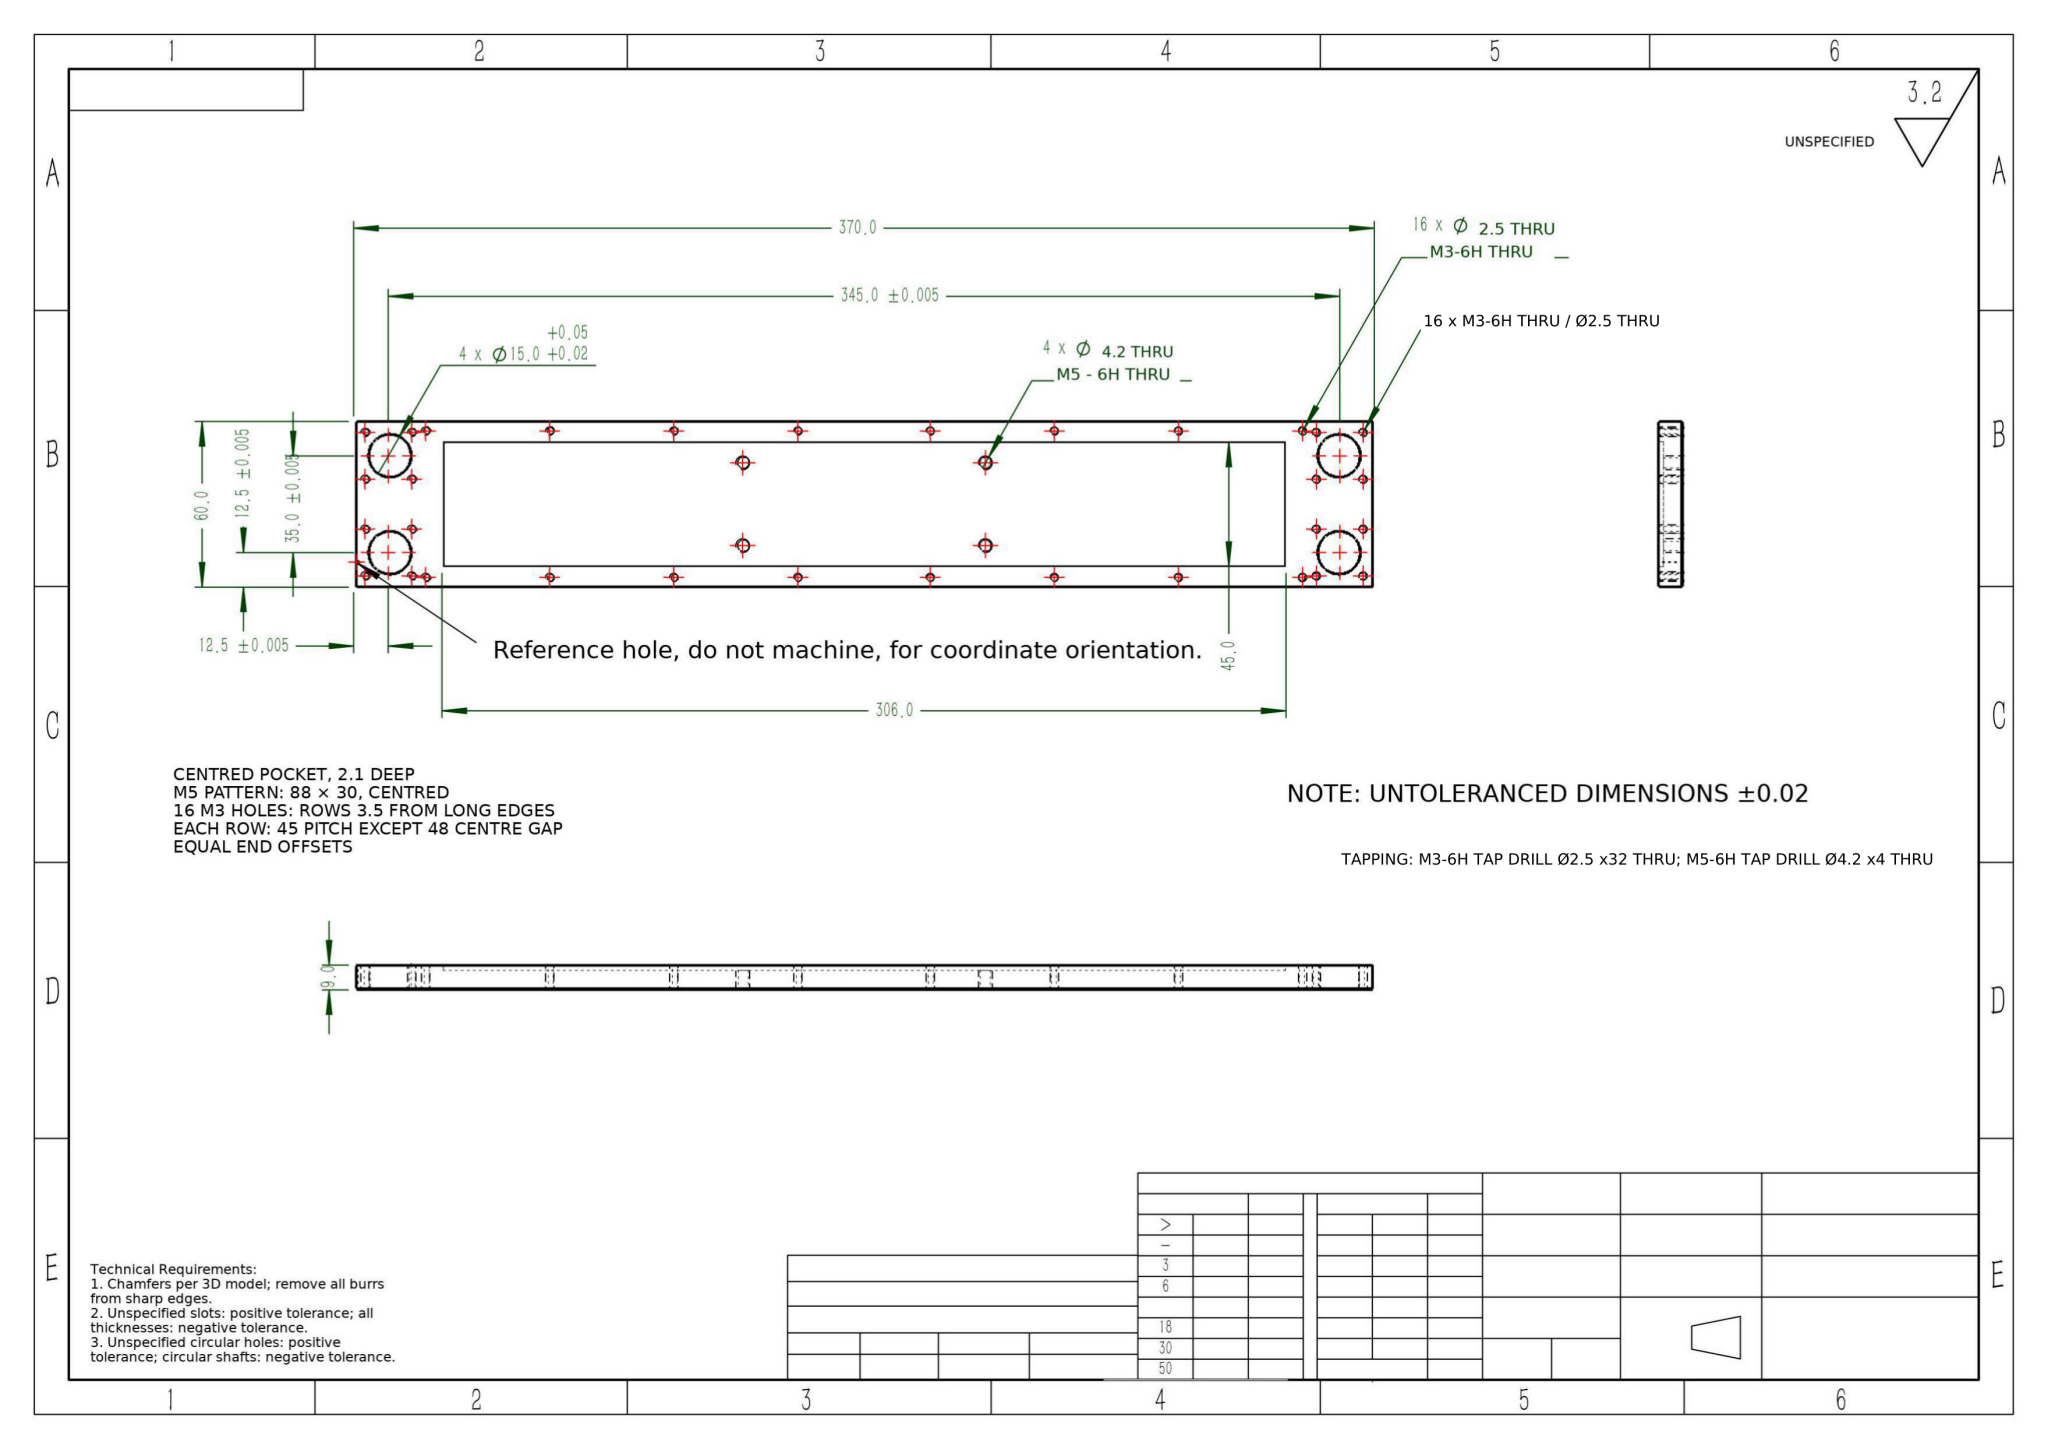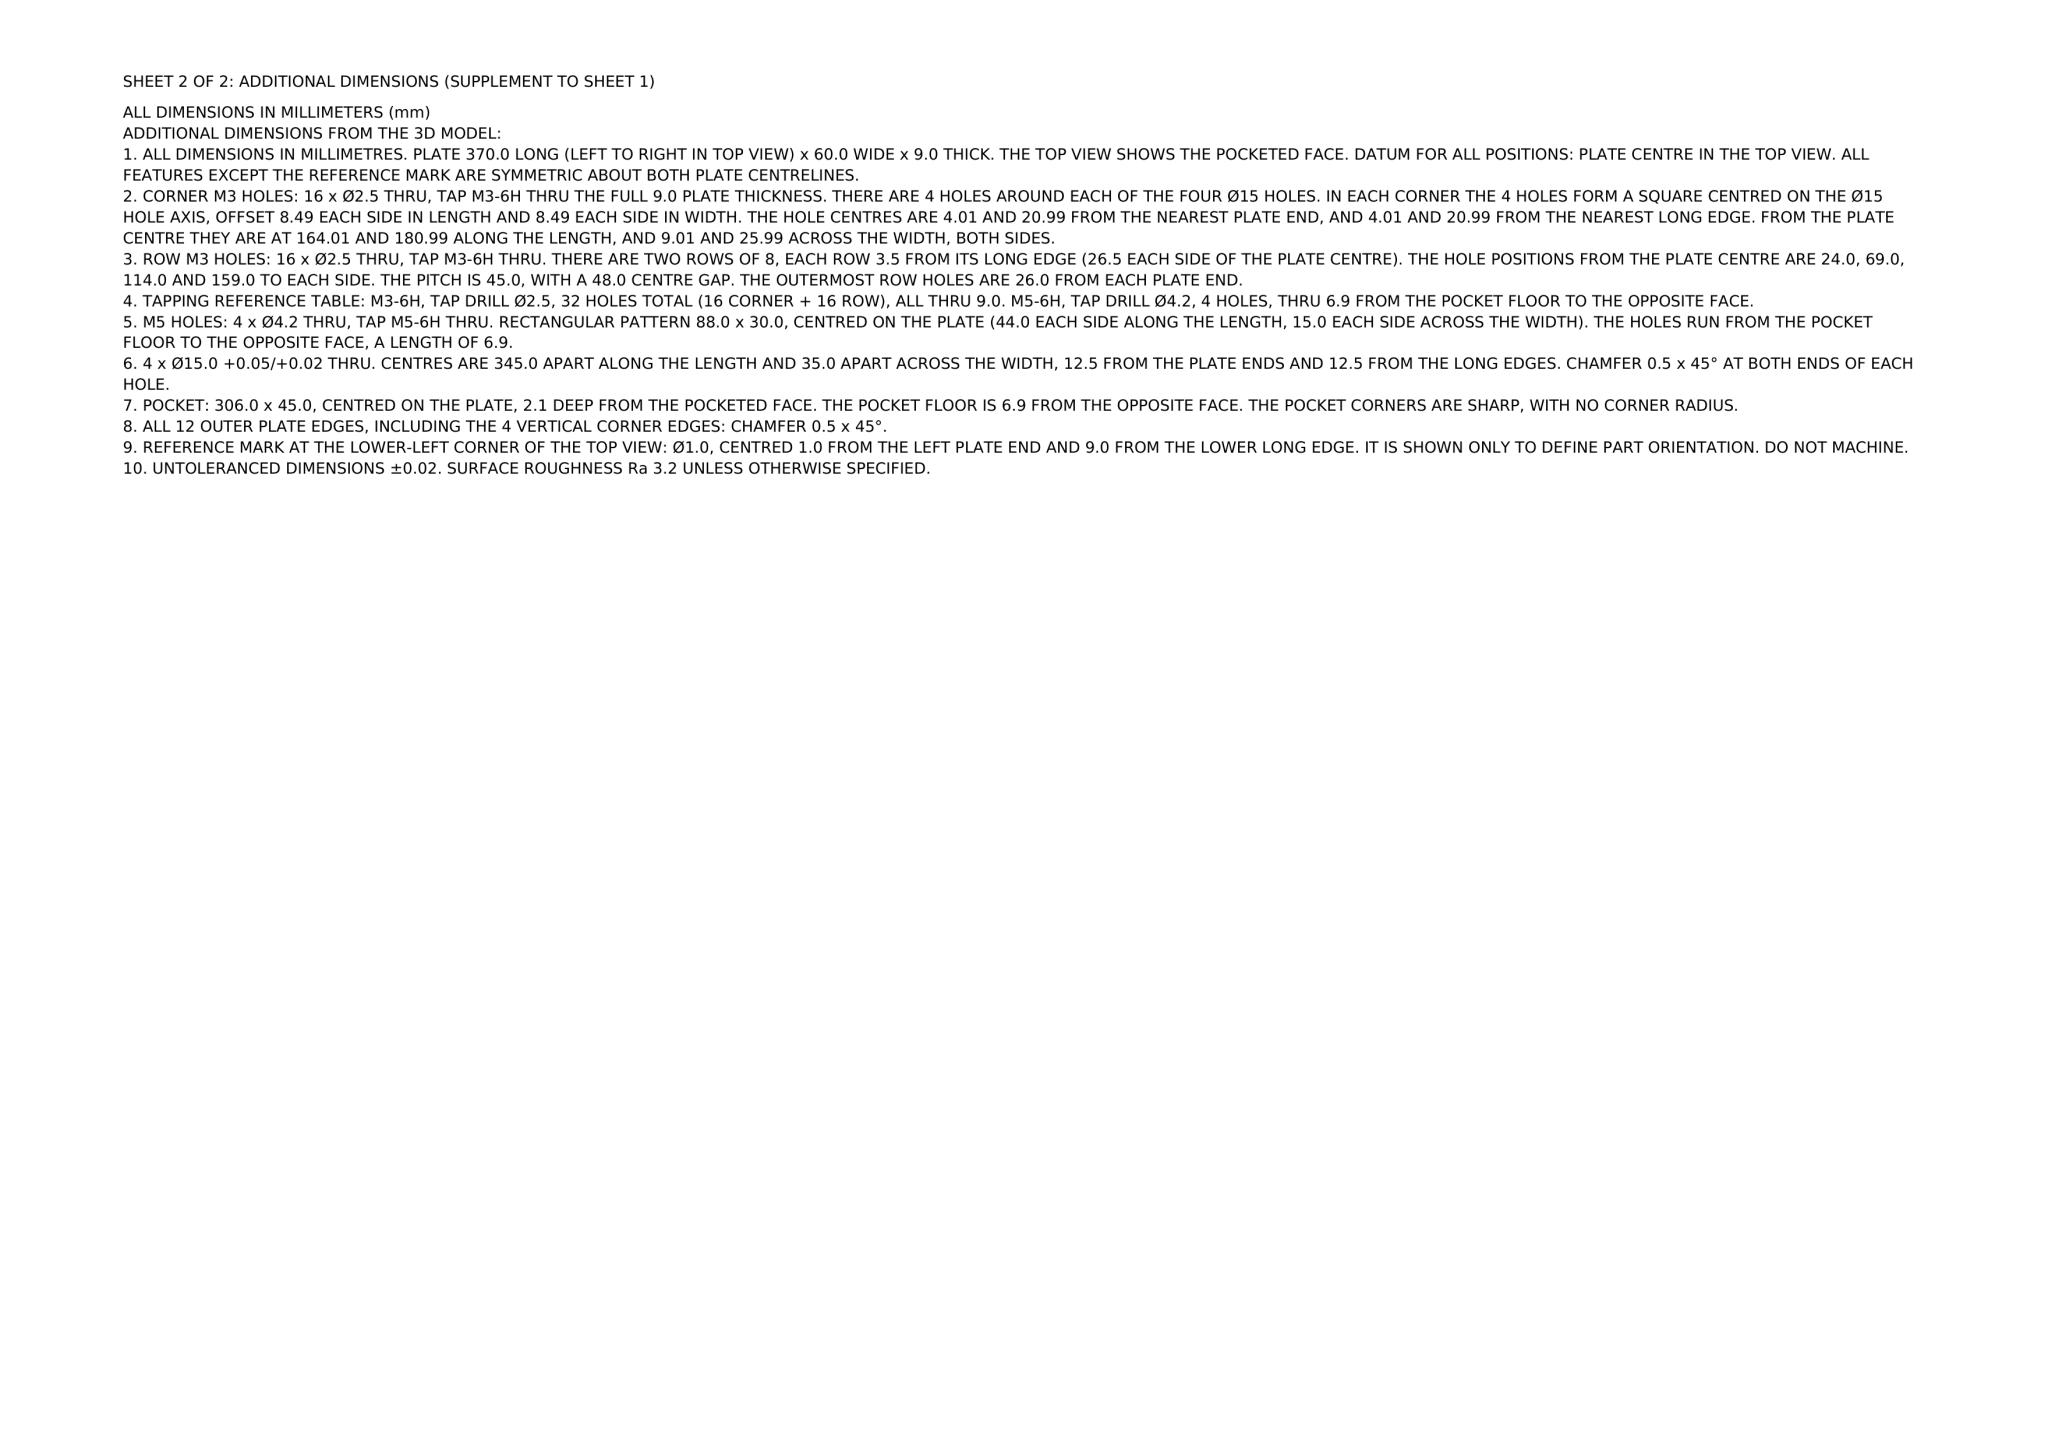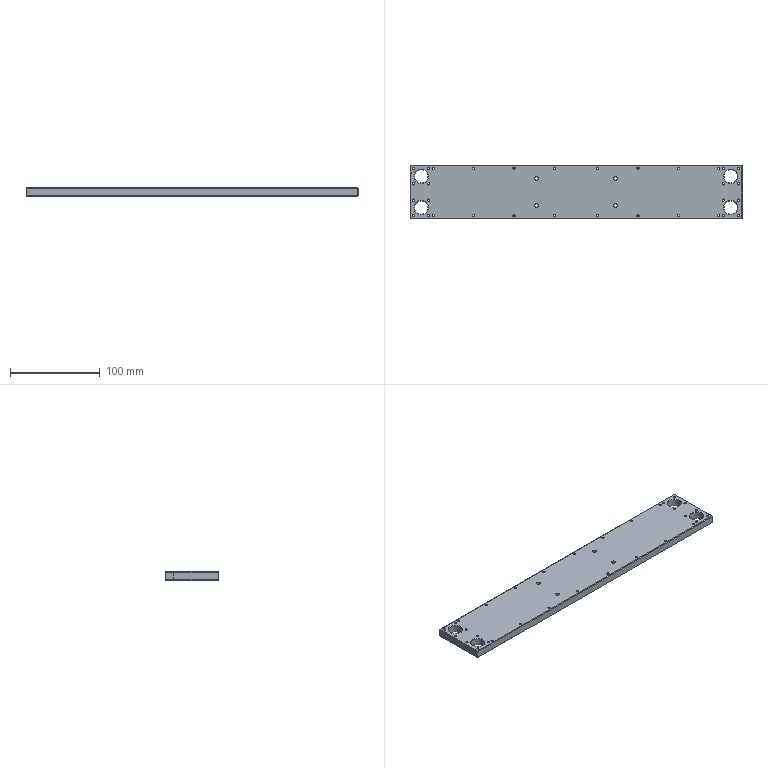Part | NX | mm | 1 solid | 129 faces | box 370 x 60 x 9 mm | volume 162451 mm3 | cylinder 82 | plane 31 | cone 16 | commonest cylinder face diameters 2.5 x64 4.2 x8 15 x8 1 x2